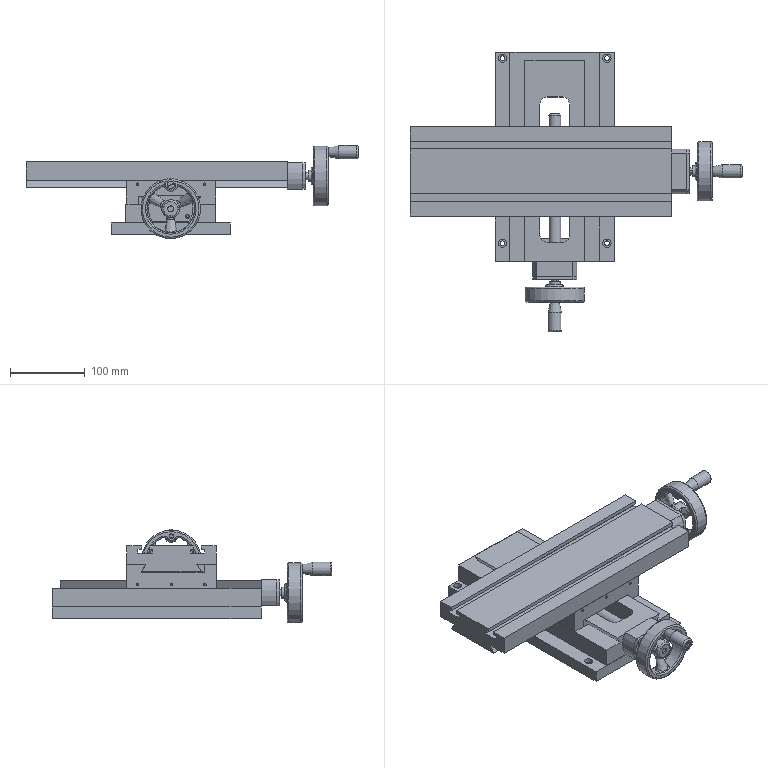Assembly | NX | mm | 22 component files | 22 solids | 449 faces | box 444.9 x 374.7 x 124.98 mm | volume 2638502 mm3 | plane 195 | cylinder 162 | cone 36 | spline 30 | torus 26 | commonest cylinder face diameters 20 x14 4.5 x14 3.3 x14 8 x12 10 x10 5 x10 6.5 x10 11 x10
Bill of materials:
unnamed part 1 | 1 |  | Housing block on a flat rectangular base flange. The raised body has chamfered upper corners and one large cylindrical through-bore running along its length. The base flange sticks out past both ends of the body and has four through-holes, one near each corner.
unnamed part 2 | 2 |  | Flanged cylindrical sleeve: a plain cylinder with a thin, larger-diameter flange at one end and a concentric through-bore.
unnamed part 3 | 2 |  | Thick block with straight top and bottom edges and convex arc-shaped ends. It has a large central through-hole and four smaller through-holes: two near each arc end, of different sizes, in an asymmetric layout.
unnamed part 4 | 1 |  | Square-ish plate or block. Its side profile has a rectangular rebate on one side and an angled (dovetail-like) rebate on the opposite side, in a C-like section. The top face has eight through-holes in a symmetric cluster (four larger, four smaller), and one side face has three small holes.
unnamed part 5 | 2 |  | Thin flat plate with straight top and bottom edges and convex arc ends. It has a large central round hole and two small through-holes at diagonally opposite positions near the arc ends.
unnamed part 6 | 1 |  | Long slender stepped cylindrical shaft. Most of its length is one main diameter. One end steps down to a smaller-diameter section with a short stepped or grooved zone and a plain end segment. The end view shows a small rectangular flat or slot feature near the outer edge.
unnamed part 7 | 1 |  | Flat rectangular plate with a large central rectangular cutout with rounded corners. It has four larger through-holes at the outer corners and six smaller through-holes around the cutout (three along each long side).
unnamed part 8 | 2 |  | Round sleeve: a cylindrical section with a rounded end, then a conical taper to a smaller-diameter flat end, with a concentric axial bore.
unnamed part 9 | 1 |  | Rectangular block with a large cylindrical through-bore and two chamfered corners on one side. One face has four small holes in a square pattern, which also appear in the opposite-face view with conical shading.
unnamed part 10 | 1 |  | Long flat bar with a constant cross-section along its length. Two undercut T-shaped slots run lengthwise in the top face, and a trapezoidal (dovetail-like) rib runs along the bottom. The end face has two small holes and a larger round feature at the center.
unnamed part 11 | 1 |  | Long slender stepped cylindrical shaft. The main body is one diameter with a shoulder down to a smaller-diameter end section that has short grooves or steps. The end view shows a small rectangular flat or slot feature near the outer edge.
unnamed part 12 | 2 |  | Three-spoke wheel. A round rim with rounded edges is joined by three tapered spokes to a central hub with a through-bore. The hub boss sticks out slightly past one face of the rim. Opposite the bottom spoke, the rim widens into a lobe on its inner edge with a small through-hole.
unnamed part 13 | 1 |  | Rectangular block with a raised dovetail-profile tongue running along its length on top. A long obround slot with rounded ends goes through it, and one end face has holes.
unnamed part 14 | 2 |  | Long straight prismatic bar with the same cross-section along its whole length. The section is a right trapezoid, with one vertical side and one angled side.
unnamed part 15 | 2 |  | Stepped round pin with a short larger-diameter head that has a straight slot across it. The middle shank steps down to a smaller-diameter end section with a chamfer.
Mates:
1. fix | base 1 component
2. concentric | base 1 edge | slide 1 edge
3. concentric | slide 1 edge | base 1 edge
4. touch align | work_table_screw 1 face | slide 1 face
5. concentric | slide_bearing_block 2 edge | slide 1 edge
6. concentric | slide_bearing_block 2 edge | slide 1 edge
7. concentric | bearing_end_cap 2 edge | slide_bearing_block 2 edge
8. concentric | bearing_end_cap 2 edge | slide_bearing_block 2 edge
9. concentric | work_table_screw 1 edge | slide_bearing_block 2 edge
10. concentric | slide_nut 1 edge | saddle 1 edge
11. concentric | slide_nut 1 edge | saddle 1 edge
12. touch align | slide_nut 1 face | work_table_screw 1 face
13. parallel | saddle 1 face | slide 1 face
14. touch align | slide_gib 2 face | saddle 1 face
15. concentric | slide_gib 2 edge | saddle 1 arc
16. concentric | slide_gib 2 edge | saddle 1 edge
17. concentric | work_table_nut 1 edge | saddle 1 edge
18. touch align | work_table_nut 1 face | slide_screw 1 face
19. touch align | work_table 1 face | slide_screw 1 face
20. concentric | bearing_end_cap 1 edge | slide_bearing_block 1 edge
21. concentric | bearing_end_cap 1 edge | slide_bearing_block 1 edge
22. concentric | work_table 1 edge | slide_bearing_block 1 edge
23. concentric | slide_bearing_block 1 edge | work_table 1 edge
24. concentric | slide_screw 1 edge | slide_bearing_block 1 edge
25. touch align | slide_gib 1 face | saddle 1 face
26. concentric | saddle 1 edge | slide_gib 1 edge
27. concentric | slide_gib 1 edge | saddle 1 edge
28. concentric | handle_bushing 2 edge | slide_screw 1 edge
29. concentric | handle_bushing 2 edge | handwheel 2 edge
30. concentric | handle 2 edge | handwheel 2 edge
31. concentric | handwheel_shaft 2 edge | handle 2 edge
32. concentric | handle 1 edge | handwheel 1 edge
33. concentric | handwheel_shaft 1 edge | handle 1 edge
34. concentric | handle_bushing 1 edge | handwheel 1 edge
35. concentric | work_table_screw 1 edge | handle_bushing 1 edge